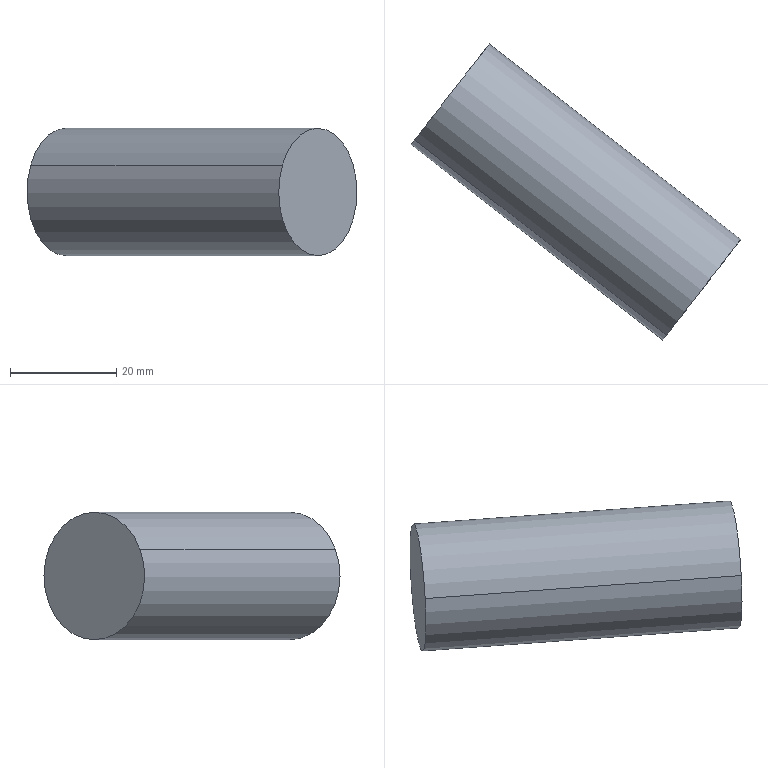Component | SolidWorks | 0803_102_Servo_Motor_850W-1_0803_Z_Servo_Motor_850W_2-1 | 1 solid | 4 faces | box 62.11 x 55.75 x 24 mm | volume 27143 mm3 | cylinder 2 | plane 2 | commonest cylinder face diameters 24 x2
build123d program:
from build123d import *

# Parameters (mm, degrees)
SKETCH1_W = 12
SKETCH1_H = 60


with BuildPart() as part:
    # Sketch1 → Revolve1 (revolve)
    with BuildSketch(Plane.XY, mode=Mode.PRIVATE) as revolve1_sk:
        with Locations((6, 30)):
            Rectangle(SKETCH1_W, SKETCH1_H)
    revolve(revolve1_sk.sketch.rotate(Axis((0, -11.341, 0), (0, 1, 0)), 90), axis=Axis((0, -11.341, 0), (0, 1, 0)))


solid = part.part

# Placed as in the assembly
solid = solid.moved(Location((-174.647, 880.212, 276.411), (-133.672, 29.313, 115.051)))
STEP:
#1=COLOUR_RGB('',0.7922,0.8196,0.9333);
#2=FILL_AREA_STYLE_COLOUR('',#1);
#3=FILL_AREA_STYLE('',(#2));
#4=SURFACE_STYLE_FILL_AREA(#3);
#5=SURFACE_SIDE_STYLE('',(#4));
#6=SURFACE_STYLE_USAGE(.BOTH.,#5);
#7=PRESENTATION_STYLE_ASSIGNMENT((#6));
#8=CARTESIAN_POINT('',(-7.138,34.316,11.082));
#9=VERTEX_POINT('',#8);
#10=CARTESIAN_POINT('',(-6.613,34.992,10.682));
#11=VERTEX_POINT('',#10);
#12=CARTESIAN_POINT('',(-6.876,34.654,10.882));
#13=DIRECTION('',(-0.7899,0.6132,0.));
#14=DIRECTION('',(-0.5555,-0.7156,0.4235));
#15=AXIS2_PLACEMENT_3D('',#12,#13,#14);
#16=CIRCLE('',#15,0.4724);
#17=EDGE_CURVE('',#9,#11,#16,.T.);
#18=ORIENTED_EDGE('',*,*,#17,.T.);
#19=CARTESIAN_POINT('',(-8.479,36.441,10.682));
#20=VERTEX_POINT('',#19);
#21=CARTESIAN_POINT('',(-8.832,36.714,10.682));
#22=DIRECTION('',(-0.7899,0.6132,0.));
#23=VECTOR('',#22,39.37);
#24=LINE('',#21,#23);
#25=EDGE_CURVE('',#11,#20,#24,.T.);
#26=ORIENTED_EDGE('',*,*,#25,.T.);
#27=CARTESIAN_POINT('',(-9.004,35.764,11.082));
#28=VERTEX_POINT('',#27);
#29=CARTESIAN_POINT('',(-8.742,36.103,10.882));
#30=DIRECTION('',(-0.7899,0.6132,0.));
#31=DIRECTION('',(-0.5555,-0.7156,0.4235));
#32=AXIS2_PLACEMENT_3D('',#29,#30,#31);
#33=CIRCLE('',#32,0.4724);
#34=EDGE_CURVE('',#28,#20,#33,.T.);
#35=ORIENTED_EDGE('',*,*,#34,.F.);
#36=CARTESIAN_POINT('',(-9.357,36.038,11.082));
#37=DIRECTION('',(-0.7899,0.6132,0.));
#38=VECTOR('',#37,39.37);
#39=LINE('',#36,#38);
#40=EDGE_CURVE('',#9,#28,#39,.T.);
#41=ORIENTED_EDGE('',*,*,#40,.F.);
#42=EDGE_LOOP('',(#18,#26,#35,#41));
#43=FACE_OUTER_BOUND('',#42,.T.);
#44=CARTESIAN_POINT('',(-9.095,36.376,10.882));
#45=DIRECTION('',(-0.7899,0.6132,0.));
#46=DIRECTION('',(-0.5555,-0.7156,0.4235));
#47=AXIS2_PLACEMENT_3D('',#44,#45,#46);
#48=CYLINDRICAL_SURFACE('',#47,0.4724);
#49=ADVANCED_FACE('',(#43),#48,.T.);
#50=ORIENTED_EDGE('',*,*,#34,.T.);
#51=CARTESIAN_POINT('',(-8.742,36.103,10.882));
#52=DIRECTION('',(-0.7899,0.6132,0.));
#53=DIRECTION('',(-0.5555,-0.7156,0.4235));
#54=AXIS2_PLACEMENT_3D('',#51,#52,#53);
#55=CIRCLE('',#54,0.4724);
#56=EDGE_CURVE('',#20,#28,#55,.T.);
#57=ORIENTED_EDGE('',*,*,#56,.T.);
#58=EDGE_LOOP('',(#50,#57));
#59=FACE_OUTER_BOUND('',#58,.T.);
#60=CARTESIAN_POINT('',(-8.742,36.103,10.882));
#61=DIRECTION('',(-0.7899,0.6132,0.));
#62=DIRECTION('',(-0.5555,-0.7156,0.4235));
#63=AXIS2_PLACEMENT_3D('',#60,#61,#62);
#64=PLANE('',#63);
#65=ADVANCED_FACE('',(#59),#64,.T.);
#66=ORIENTED_EDGE('',*,*,#25,.F.);
#67=CARTESIAN_POINT('',(-6.876,34.654,10.882));
#68=DIRECTION('',(-0.7899,0.6132,0.));
#69=DIRECTION('',(-0.5555,-0.7156,0.4235));
#70=AXIS2_PLACEMENT_3D('',#67,#68,#69);
#71=CIRCLE('',#70,0.4724);
#72=EDGE_CURVE('',#11,#9,#71,.T.);
#73=ORIENTED_EDGE('',*,*,#72,.T.);
#74=ORIENTED_EDGE('',*,*,#40,.T.);
#75=ORIENTED_EDGE('',*,*,#56,.F.);
#76=EDGE_LOOP('',(#66,#73,#74,#75));
#77=FACE_OUTER_BOUND('',#76,.T.);
#78=CARTESIAN_POINT('',(-9.095,36.376,10.882));
#79=DIRECTION('',(-0.7899,0.6132,0.));
#80=DIRECTION('',(-0.5555,-0.7156,0.4235));
#81=AXIS2_PLACEMENT_3D('',#78,#79,#80);
#82=CYLINDRICAL_SURFACE('',#81,0.4724);
#83=ADVANCED_FACE('',(#77),#82,.T.);
#84=ORIENTED_EDGE('',*,*,#17,.F.);
#85=ORIENTED_EDGE('',*,*,#72,.F.);
#86=EDGE_LOOP('',(#84,#85));
#87=FACE_OUTER_BOUND('',#86,.T.);
#88=CARTESIAN_POINT('',(-6.876,34.654,10.882));
#89=DIRECTION('',(0.7899,-0.6132,-0.));
#90=DIRECTION('',(0.5555,0.7156,-0.4235));
#91=AXIS2_PLACEMENT_3D('',#88,#89,#90);
#92=PLANE('',#91);
#93=ADVANCED_FACE('',(#87),#92,.T.);
#94=CLOSED_SHELL('',(#49,#65,#83,#93));
#95=MANIFOLD_SOLID_BREP('',#94);
#96=STYLED_ITEM('',(#7),#95);
#97=PRESENTATION_LAYER_ASSIGNMENT('','',(#96));
#98=(LENGTH_UNIT()NAMED_UNIT(*)SI_UNIT($,.METRE.));
#99=LENGTH_MEASURE_WITH_UNIT(LENGTH_MEASURE(0.0254),#98);
#100=DIMENSIONAL_EXPONENTS(1.,0.,0.,0.,0.,0.,0.);
#101=(CONVERSION_BASED_UNIT('',#99)LENGTH_UNIT()NAMED_UNIT(#100));
#102=UNCERTAINTY_MEASURE_WITH_UNIT(LENGTH_MEASURE(0.00001),#101,'','');
#103=(NAMED_UNIT(*)PLANE_ANGLE_UNIT()SI_UNIT($,.RADIAN.));
#104=(NAMED_UNIT(*)SI_UNIT($,.STERADIAN.)SOLID_ANGLE_UNIT());
#105=(GEOMETRIC_REPRESENTATION_CONTEXT(3)GLOBAL_UNCERTAINTY_ASSIGNED_CONTEXT((#102))GLOBAL_UNIT_ASSIGNED_CONTEXT((#101,#103,#104))REPRESENTATION_CONTEXT('',''));
#106=MECHANICAL_DESIGN_GEOMETRIC_PRESENTATION_REPRESENTATION('',(#96),#105);
#107=CARTESIAN_POINT('',(0.,0.,0.));
#108=DIRECTION('',(0.,0.,1.));
#109=DIRECTION('',(1.,0.,0.));
#110=AXIS2_PLACEMENT_3D('',#107,#108,#109);
#111=(LENGTH_UNIT()NAMED_UNIT(*)SI_UNIT($,.METRE.));
#112=LENGTH_MEASURE_WITH_UNIT(LENGTH_MEASURE(0.0254),#111);
#113=DIMENSIONAL_EXPONENTS(1.,0.,0.,0.,0.,0.,0.);
#114=(CONVERSION_BASED_UNIT('',#112)LENGTH_UNIT()NAMED_UNIT(#113));
#115=UNCERTAINTY_MEASURE_WITH_UNIT(LENGTH_MEASURE(0.00001),#114,'','');
#116=(NAMED_UNIT(*)PLANE_ANGLE_UNIT()SI_UNIT($,.RADIAN.));
#117=(NAMED_UNIT(*)SI_UNIT($,.STERADIAN.)SOLID_ANGLE_UNIT());
#118=(GEOMETRIC_REPRESENTATION_CONTEXT(3)GLOBAL_UNCERTAINTY_ASSIGNED_CONTEXT((#115))GLOBAL_UNIT_ASSIGNED_CONTEXT((#114,#116,#117))REPRESENTATION_CONTEXT('',''));
#119=ADVANCED_BREP_SHAPE_REPRESENTATION('',(#95,#110),#118);